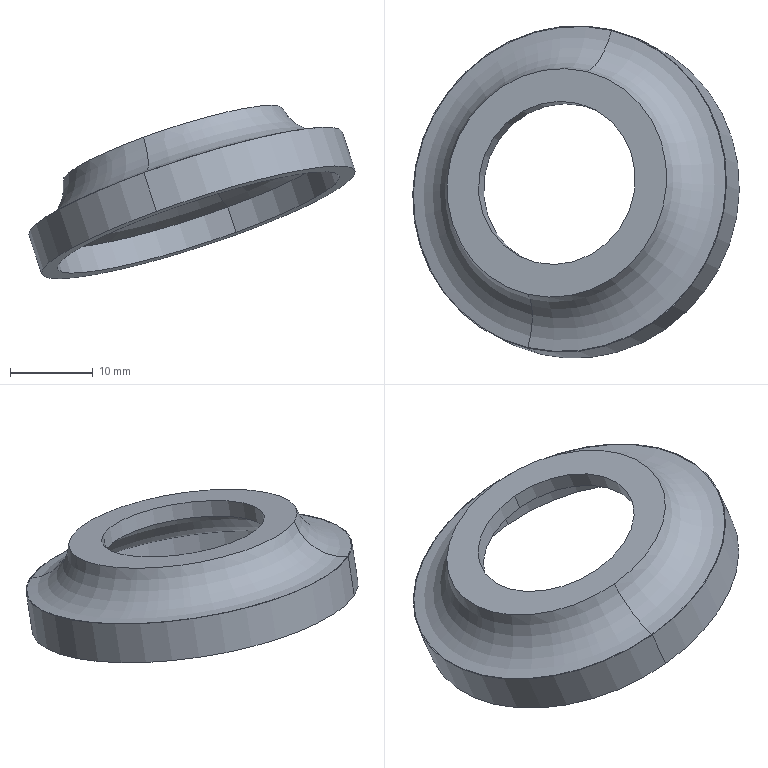Component | SolidWorks | FilmPressingSoilCoveringMechanism2Reverse-2_AttachedSoilDiskAssembly2-1_DustCover-1 | 1 solid | 14 faces | box 39.58 x 40.3 x 21.03 mm | volume 3029 mm3 | cylinder 6 | torus 4 | plane 4 | commonest cylinder face diameters 20 x2 36 x2 40 x2
STEP:
#1=COLOUR_RGB('',0.7922,0.8196,0.9333);
#2=FILL_AREA_STYLE_COLOUR('',#1);
#3=FILL_AREA_STYLE('',(#2));
#4=SURFACE_STYLE_FILL_AREA(#3);
#5=SURFACE_SIDE_STYLE('',(#4));
#6=SURFACE_STYLE_USAGE(.BOTH.,#5);
#7=PRESENTATION_STYLE_ASSIGNMENT((#6));
#8=CARTESIAN_POINT('',(-76.149,-11.265,104.072));
#9=VERTEX_POINT('',#8);
#10=CARTESIAN_POINT('',(-76.349,-12.025,104.124));
#11=VERTEX_POINT('',#10);
#12=CARTESIAN_POINT('',(-76.249,-11.645,104.098));
#13=DIRECTION('',(-0.3093,0.1459,0.9397));
#14=DIRECTION('',(-0.2542,-0.9649,0.06614));
#15=AXIS2_PLACEMENT_3D('',#12,#13,#14);
#16=CIRCLE('',#15,0.3937);
#17=EDGE_CURVE('',#9,#11,#16,.T.);
#18=ORIENTED_EDGE('',*,*,#17,.F.);
#19=CARTESIAN_POINT('',(-76.173,-11.254,104.146));
#20=VERTEX_POINT('',#19);
#21=CARTESIAN_POINT('',(-76.027,-11.323,103.702));
#22=DIRECTION('',(-0.3093,0.1459,0.9397));
#23=VECTOR('',#22,39.37);
#24=LINE('',#21,#23);
#25=EDGE_CURVE('',#9,#20,#24,.T.);
#26=ORIENTED_EDGE('',*,*,#25,.T.);
#27=CARTESIAN_POINT('',(-76.374,-12.013,104.198));
#28=VERTEX_POINT('',#27);
#29=CARTESIAN_POINT('',(-76.273,-11.634,104.172));
#30=DIRECTION('',(-0.3093,0.1459,0.9397));
#31=DIRECTION('',(-0.2542,-0.9649,0.06614));
#32=AXIS2_PLACEMENT_3D('',#29,#30,#31);
#33=CIRCLE('',#32,0.3937);
#34=EDGE_CURVE('',#20,#28,#33,.T.);
#35=ORIENTED_EDGE('',*,*,#34,.T.);
#36=CARTESIAN_POINT('',(-76.227,-12.082,103.754));
#37=DIRECTION('',(-0.3093,0.1459,0.9397));
#38=VECTOR('',#37,39.37);
#39=LINE('',#36,#38);
#40=EDGE_CURVE('',#11,#28,#39,.T.);
#41=ORIENTED_EDGE('',*,*,#40,.F.);
#42=EDGE_LOOP('',(#18,#26,#35,#41));
#43=FACE_OUTER_BOUND('',#42,.T.);
#44=CARTESIAN_POINT('',(-76.127,-11.703,103.728));
#45=DIRECTION('',(-0.3093,0.1459,0.9397));
#46=DIRECTION('',(-0.2542,-0.9649,0.06614));
#47=AXIS2_PLACEMENT_3D('',#44,#45,#46);
#48=CYLINDRICAL_SURFACE('',#47,0.3937);
#49=ADVANCED_FACE('',(#43),#48,.F.);
#50=CARTESIAN_POINT('',(-76.374,-12.12,104.13));
#51=VERTEX_POINT('',#50);
#52=CARTESIAN_POINT('',(-76.124,-11.17,104.065));
#53=VERTEX_POINT('',#52);
#54=CARTESIAN_POINT('',(-76.249,-11.645,104.098));
#55=DIRECTION('',(-0.3093,0.1459,0.9397));
#56=DIRECTION('',(0.2542,0.9649,-0.06614));
#57=AXIS2_PLACEMENT_3D('',#54,#55,#56);
#58=CIRCLE('',#57,0.4921);
#59=EDGE_CURVE('',#51,#53,#58,.T.);
#60=ORIENTED_EDGE('',*,*,#59,.T.);
#61=CARTESIAN_POINT('',(-76.011,-10.989,103.875));
#62=VERTEX_POINT('',#61);
#63=CARTESIAN_POINT('',(-76.086,-10.871,104.157));
#64=DIRECTION('',(0.9163,-0.2184,0.3356));
#65=DIRECTION('',(0.3439,0.,-0.939));
#66=AXIS2_PLACEMENT_3D('',#63,#64,#65);
#67=CIRCLE('',#66,0.315);
#68=EDGE_CURVE('',#53,#62,#67,.T.);
#69=ORIENTED_EDGE('',*,*,#68,.T.);
#70=CARTESIAN_POINT('',(-76.371,-12.356,103.968));
#71=VERTEX_POINT('',#70);
#72=CARTESIAN_POINT('',(-76.191,-11.672,103.922));
#73=DIRECTION('',(0.3093,-0.1459,-0.9397));
#74=DIRECTION('',(-0.2542,-0.9649,0.06614));
#75=AXIS2_PLACEMENT_3D('',#72,#73,#74);
#76=CIRCLE('',#75,0.7087);
#77=EDGE_CURVE('',#62,#71,#76,.T.);
#78=ORIENTED_EDGE('',*,*,#77,.T.);
#79=CARTESIAN_POINT('',(-76.485,-12.384,104.261));
#80=DIRECTION('',(-0.9163,0.2184,-0.3356));
#81=DIRECTION('',(-0.3439,0.,0.939));
#82=AXIS2_PLACEMENT_3D('',#79,#80,#81);
#83=CIRCLE('',#82,0.315);
#84=EDGE_CURVE('',#51,#71,#83,.T.);
#85=ORIENTED_EDGE('',*,*,#84,.F.);
#86=EDGE_LOOP('',(#60,#69,#78,#85));
#87=FACE_OUTER_BOUND('',#86,.T.);
#88=CARTESIAN_POINT('',(-76.286,-11.628,104.209));
#89=DIRECTION('',(-0.3093,0.1459,0.9397));
#90=DIRECTION('',(-0.2542,-0.9649,0.06614));
#91=AXIS2_PLACEMENT_3D('',#88,#89,#90);
#92=TOROIDAL_SURFACE('',#91,0.7841,0.315);
#93=ADVANCED_FACE('',(#87),#92,.T.);
#94=CARTESIAN_POINT('',(-76.191,-11.672,103.922));
#95=DIRECTION('',(0.3093,-0.1459,-0.9397));
#96=DIRECTION('',(-0.2542,-0.9649,0.06614));
#97=AXIS2_PLACEMENT_3D('',#94,#95,#96);
#98=CIRCLE('',#97,0.7087);
#99=EDGE_CURVE('',#71,#62,#98,.T.);
#100=ORIENTED_EDGE('',*,*,#99,.F.);
#101=CARTESIAN_POINT('',(-76.332,-12.375,103.849));
#102=VERTEX_POINT('',#101);
#103=CARTESIAN_POINT('',(-76.393,-12.346,104.034));
#104=DIRECTION('',(0.3093,-0.1459,-0.9397));
#105=VECTOR('',#104,39.37);
#106=LINE('',#103,#105);
#107=EDGE_CURVE('',#71,#102,#106,.T.);
#108=ORIENTED_EDGE('',*,*,#107,.T.);
#109=CARTESIAN_POINT('',(-75.972,-11.007,103.755));
#110=VERTEX_POINT('',#109);
#111=CARTESIAN_POINT('',(-76.152,-11.691,103.802));
#112=DIRECTION('',(-0.3093,0.1459,0.9397));
#113=DIRECTION('',(-0.2542,-0.9649,0.06614));
#114=AXIS2_PLACEMENT_3D('',#111,#112,#113);
#115=CIRCLE('',#114,0.7087);
#116=EDGE_CURVE('',#110,#102,#115,.T.);
#117=ORIENTED_EDGE('',*,*,#116,.F.);
#118=CARTESIAN_POINT('',(-76.032,-10.979,103.94));
#119=DIRECTION('',(0.3093,-0.1459,-0.9397));
#120=VECTOR('',#119,39.37);
#121=LINE('',#118,#120);
#122=EDGE_CURVE('',#62,#110,#121,.T.);
#123=ORIENTED_EDGE('',*,*,#122,.F.);
#124=EDGE_LOOP('',(#100,#108,#117,#123));
#125=FACE_OUTER_BOUND('',#124,.T.);
#126=CARTESIAN_POINT('',(-76.213,-11.662,103.987));
#127=DIRECTION('',(0.3093,-0.1459,-0.9397));
#128=DIRECTION('',(0.2542,0.9649,-0.06614));
#129=AXIS2_PLACEMENT_3D('',#126,#127,#128);
#130=CYLINDRICAL_SURFACE('',#129,0.7087);
#131=ADVANCED_FACE('',(#125),#130,.F.);
#132=CARTESIAN_POINT('',(-76.133,-11.102,104.135));
#133=VERTEX_POINT('',#132);
#134=CARTESIAN_POINT('',(-76.414,-12.165,104.208));
#135=VERTEX_POINT('',#134);
#136=CARTESIAN_POINT('',(-76.273,-11.634,104.172));
#137=DIRECTION('',(-0.3093,0.1459,0.9397));
#138=DIRECTION('',(-0.2542,-0.9649,0.06614));
#139=AXIS2_PLACEMENT_3D('',#136,#137,#138);
#140=CIRCLE('',#139,0.5512);
#141=EDGE_CURVE('',#133,#135,#140,.T.);
#142=ORIENTED_EDGE('',*,*,#141,.F.);
#143=CARTESIAN_POINT('',(-76.013,-10.906,103.935));
#144=VERTEX_POINT('',#143);
#145=CARTESIAN_POINT('',(-76.086,-10.871,104.157));
#146=DIRECTION('',(0.9163,-0.2184,0.3356));
#147=DIRECTION('',(0.3439,0.,-0.939));
#148=AXIS2_PLACEMENT_3D('',#145,#146,#147);
#149=CIRCLE('',#148,0.2362);
#150=EDGE_CURVE('',#133,#144,#149,.T.);
#151=ORIENTED_EDGE('',*,*,#150,.T.);
#152=CARTESIAN_POINT('',(-76.412,-12.419,104.039));
#153=VERTEX_POINT('',#152);
#154=CARTESIAN_POINT('',(-76.213,-11.662,103.987));
#155=DIRECTION('',(0.3093,-0.1459,-0.9397));
#156=DIRECTION('',(-0.2542,-0.9649,0.06614));
#157=AXIS2_PLACEMENT_3D('',#154,#155,#156);
#158=CIRCLE('',#157,0.7841);
#159=EDGE_CURVE('',#153,#144,#158,.T.);
#160=ORIENTED_EDGE('',*,*,#159,.F.);
#161=CARTESIAN_POINT('',(-76.485,-12.384,104.261));
#162=DIRECTION('',(-0.9163,0.2184,-0.3356));
#163=DIRECTION('',(-0.3439,0.,0.939));
#164=AXIS2_PLACEMENT_3D('',#161,#162,#163);
#165=CIRCLE('',#164,0.2362);
#166=EDGE_CURVE('',#135,#153,#165,.T.);
#167=ORIENTED_EDGE('',*,*,#166,.F.);
#168=EDGE_LOOP('',(#142,#151,#160,#167));
#169=FACE_OUTER_BOUND('',#168,.T.);
#170=CARTESIAN_POINT('',(-76.286,-11.628,104.209));
#171=DIRECTION('',(-0.3093,0.1459,0.9397));
#172=DIRECTION('',(-0.2542,-0.9649,0.06614));
#173=AXIS2_PLACEMENT_3D('',#170,#171,#172);
#174=TOROIDAL_SURFACE('',#173,0.7841,0.2362);
#175=ADVANCED_FACE('',(#169),#174,.F.);
#176=CARTESIAN_POINT('',(-76.413,-12.422,104.039));
#177=VERTEX_POINT('',#176);
#178=CARTESIAN_POINT('',(-76.012,-10.903,103.935));
#179=VERTEX_POINT('',#178);
#180=CARTESIAN_POINT('',(-76.213,-11.662,103.987));
#181=DIRECTION('',(-0.3093,0.1459,0.9397));
#182=DIRECTION('',(-0.2542,-0.9649,0.06614));
#183=AXIS2_PLACEMENT_3D('',#180,#181,#182);
#184=CIRCLE('',#183,0.7874);
#185=EDGE_CURVE('',#177,#179,#184,.T.);
#186=ORIENTED_EDGE('',*,*,#185,.F.);
#187=CARTESIAN_POINT('',(-76.352,-12.451,103.854));
#188=VERTEX_POINT('',#187);
#189=CARTESIAN_POINT('',(-76.413,-12.422,104.039));
#190=DIRECTION('',(0.3093,-0.1459,-0.9397));
#191=VECTOR('',#190,39.37);
#192=LINE('',#189,#191);
#193=EDGE_CURVE('',#177,#188,#192,.T.);
#194=ORIENTED_EDGE('',*,*,#193,.T.);
#195=CARTESIAN_POINT('',(-75.952,-10.931,103.75));
#196=VERTEX_POINT('',#195);
#197=CARTESIAN_POINT('',(-76.152,-11.691,103.802));
#198=DIRECTION('',(-0.3093,0.1459,0.9397));
#199=DIRECTION('',(-0.2542,-0.9649,0.06614));
#200=AXIS2_PLACEMENT_3D('',#197,#198,#199);
#201=CIRCLE('',#200,0.7874);
#202=EDGE_CURVE('',#188,#196,#201,.T.);
#203=ORIENTED_EDGE('',*,*,#202,.T.);
#204=CARTESIAN_POINT('',(-76.012,-10.903,103.935));
#205=DIRECTION('',(0.3093,-0.1459,-0.9397));
#206=VECTOR('',#205,39.37);
#207=LINE('',#204,#206);
#208=EDGE_CURVE('',#179,#196,#207,.T.);
#209=ORIENTED_EDGE('',*,*,#208,.F.);
#210=EDGE_LOOP('',(#186,#194,#203,#209));
#211=FACE_OUTER_BOUND('',#210,.T.);
#212=CARTESIAN_POINT('',(-76.213,-11.662,103.987));
#213=DIRECTION('',(0.3093,-0.1459,-0.9397));
#214=DIRECTION('',(0.2542,0.9649,-0.06614));
#215=AXIS2_PLACEMENT_3D('',#212,#213,#214);
#216=CYLINDRICAL_SURFACE('',#215,0.7874);
#217=ADVANCED_FACE('',(#211),#216,.T.);
#218=ORIENTED_EDGE('',*,*,#159,.T.);
#219=CARTESIAN_POINT('',(-76.213,-11.662,103.987));
#220=DIRECTION('',(0.3093,-0.1459,-0.9397));
#221=DIRECTION('',(-0.2542,-0.9649,0.06614));
#222=AXIS2_PLACEMENT_3D('',#219,#220,#221);
#223=CIRCLE('',#222,0.7841);
#224=EDGE_CURVE('',#144,#153,#223,.T.);
#225=ORIENTED_EDGE('',*,*,#224,.T.);
#226=EDGE_LOOP('',(#218,#225));
#227=FACE_BOUND('',#226,.T.);
#228=CARTESIAN_POINT('',(-76.213,-11.662,103.987));
#229=DIRECTION('',(-0.3093,0.1459,0.9397));
#230=DIRECTION('',(-0.2542,-0.9649,0.06614));
#231=AXIS2_PLACEMENT_3D('',#228,#229,#230);
#232=CIRCLE('',#231,0.7874);
#233=EDGE_CURVE('',#179,#177,#232,.T.);
#234=ORIENTED_EDGE('',*,*,#233,.T.);
#235=ORIENTED_EDGE('',*,*,#185,.T.);
#236=EDGE_LOOP('',(#234,#235));
#237=FACE_OUTER_BOUND('',#236,.T.);
#238=CARTESIAN_POINT('',(-76.213,-11.662,103.987));
#239=DIRECTION('',(-0.3093,0.1459,0.9397));
#240=DIRECTION('',(-0.2542,-0.9649,0.06614));
#241=AXIS2_PLACEMENT_3D('',#238,#239,#240);
#242=PLANE('',#241);
#243=ADVANCED_FACE('',(#227,#237),#242,.T.);
#244=ORIENTED_EDGE('',*,*,#193,.F.);
#245=ORIENTED_EDGE('',*,*,#233,.F.);
#246=ORIENTED_EDGE('',*,*,#208,.T.);
#247=CARTESIAN_POINT('',(-76.152,-11.691,103.802));
#248=DIRECTION('',(-0.3093,0.1459,0.9397));
#249=DIRECTION('',(-0.2542,-0.9649,0.06614));
#250=AXIS2_PLACEMENT_3D('',#247,#248,#249);
#251=CIRCLE('',#250,0.7874);
#252=EDGE_CURVE('',#196,#188,#251,.T.);
#253=ORIENTED_EDGE('',*,*,#252,.T.);
#254=EDGE_LOOP('',(#244,#245,#246,#253));
#255=FACE_OUTER_BOUND('',#254,.T.);
#256=CARTESIAN_POINT('',(-76.213,-11.662,103.987));
#257=DIRECTION('',(0.3093,-0.1459,-0.9397));
#258=DIRECTION('',(0.2542,0.9649,-0.06614));
#259=AXIS2_PLACEMENT_3D('',#256,#257,#258);
#260=CYLINDRICAL_SURFACE('',#259,0.7874);
#261=ADVANCED_FACE('',(#255),#260,.T.);
#262=ORIENTED_EDGE('',*,*,#116,.T.);
#263=CARTESIAN_POINT('',(-76.152,-11.691,103.802));
#264=DIRECTION('',(-0.3093,0.1459,0.9397));
#265=DIRECTION('',(-0.2542,-0.9649,0.06614));
#266=AXIS2_PLACEMENT_3D('',#263,#264,#265);
#267=CIRCLE('',#266,0.7087);
#268=EDGE_CURVE('',#102,#110,#267,.T.);
#269=ORIENTED_EDGE('',*,*,#268,.T.);
#270=EDGE_LOOP('',(#262,#269));
#271=FACE_BOUND('',#270,.T.);
#272=ORIENTED_EDGE('',*,*,#252,.F.);
#273=ORIENTED_EDGE('',*,*,#202,.F.);
#274=EDGE_LOOP('',(#272,#273));
#275=FACE_OUTER_BOUND('',#274,.T.);
#276=CARTESIAN_POINT('',(-76.152,-11.691,103.802));
#277=DIRECTION('',(-0.3093,0.1459,0.9397));
#278=DIRECTION('',(-0.2542,-0.9649,0.06614));
#279=AXIS2_PLACEMENT_3D('',#276,#277,#278);
#280=PLANE('',#279);
#281=ADVANCED_FACE('',(#271,#275),#280,.F.);
#282=CARTESIAN_POINT('',(-76.273,-11.634,104.172));
#283=DIRECTION('',(-0.3093,0.1459,0.9397));
#284=DIRECTION('',(-0.2542,-0.9649,0.06614));
#285=AXIS2_PLACEMENT_3D('',#282,#283,#284);
#286=CIRCLE('',#285,0.3937);
#287=EDGE_CURVE('',#28,#20,#286,.T.);
#288=ORIENTED_EDGE('',*,*,#287,.F.);
#289=ORIENTED_EDGE('',*,*,#34,.F.);
#290=EDGE_LOOP('',(#288,#289));
#291=FACE_BOUND('',#290,.T.);
#292=CARTESIAN_POINT('',(-76.273,-11.634,104.172));
#293=DIRECTION('',(-0.3093,0.1459,0.9397));
#294=DIRECTION('',(-0.2542,-0.9649,0.06614));
#295=AXIS2_PLACEMENT_3D('',#292,#293,#294);
#296=CIRCLE('',#295,0.5512);
#297=EDGE_CURVE('',#135,#133,#296,.T.);
#298=ORIENTED_EDGE('',*,*,#297,.T.);
#299=ORIENTED_EDGE('',*,*,#141,.T.);
#300=EDGE_LOOP('',(#298,#299));
#301=FACE_OUTER_BOUND('',#300,.T.);
#302=CARTESIAN_POINT('',(-76.273,-11.634,104.172));
#303=DIRECTION('',(-0.3093,0.1459,0.9397));
#304=DIRECTION('',(-0.2542,-0.9649,0.06614));
#305=AXIS2_PLACEMENT_3D('',#302,#303,#304);
#306=PLANE('',#305);
#307=ADVANCED_FACE('',(#291,#301),#306,.T.);
#308=ORIENTED_EDGE('',*,*,#150,.F.);
#309=ORIENTED_EDGE('',*,*,#297,.F.);
#310=ORIENTED_EDGE('',*,*,#166,.T.);
#311=ORIENTED_EDGE('',*,*,#224,.F.);
#312=EDGE_LOOP('',(#308,#309,#310,#311));
#313=FACE_OUTER_BOUND('',#312,.T.);
#314=CARTESIAN_POINT('',(-76.286,-11.628,104.209));
#315=DIRECTION('',(-0.3093,0.1459,0.9397));
#316=DIRECTION('',(-0.2542,-0.9649,0.06614));
#317=AXIS2_PLACEMENT_3D('',#314,#315,#316);
#318=TOROIDAL_SURFACE('',#317,0.7841,0.2362);
#319=ADVANCED_FACE('',(#313),#318,.F.);
#320=ORIENTED_EDGE('',*,*,#107,.F.);
#321=ORIENTED_EDGE('',*,*,#77,.F.);
#322=ORIENTED_EDGE('',*,*,#122,.T.);
#323=ORIENTED_EDGE('',*,*,#268,.F.);
#324=EDGE_LOOP('',(#320,#321,#322,#323));
#325=FACE_OUTER_BOUND('',#324,.T.);
#326=CARTESIAN_POINT('',(-76.213,-11.662,103.987));
#327=DIRECTION('',(0.3093,-0.1459,-0.9397));
#328=DIRECTION('',(0.2542,0.9649,-0.06614));
#329=AXIS2_PLACEMENT_3D('',#326,#327,#328);
#330=CYLINDRICAL_SURFACE('',#329,0.7087);
#331=ADVANCED_FACE('',(#325),#330,.F.);
#332=CARTESIAN_POINT('',(-76.249,-11.645,104.098));
#333=DIRECTION('',(-0.3093,0.1459,0.9397));
#334=DIRECTION('',(-0.2542,-0.9649,0.06614));
#335=AXIS2_PLACEMENT_3D('',#332,#333,#334);
#336=CIRCLE('',#335,0.3937);
#337=EDGE_CURVE('',#11,#9,#336,.T.);
#338=ORIENTED_EDGE('',*,*,#337,.T.);
#339=ORIENTED_EDGE('',*,*,#17,.T.);
#340=EDGE_LOOP('',(#338,#339));
#341=FACE_BOUND('',#340,.T.);
#342=ORIENTED_EDGE('',*,*,#59,.F.);
#343=CARTESIAN_POINT('',(-76.249,-11.645,104.098));
#344=DIRECTION('',(-0.3093,0.1459,0.9397));
#345=DIRECTION('',(0.2542,0.9649,-0.06614));
#346=AXIS2_PLACEMENT_3D('',#343,#344,#345);
#347=CIRCLE('',#346,0.4921);
#348=EDGE_CURVE('',#53,#51,#347,.T.);
#349=ORIENTED_EDGE('',*,*,#348,.F.);
#350=EDGE_LOOP('',(#342,#349));
#351=FACE_OUTER_BOUND('',#350,.T.);
#352=CARTESIAN_POINT('',(-76.249,-11.645,104.098));
#353=DIRECTION('',(-0.3093,0.1459,0.9397));
#354=DIRECTION('',(-0.2542,-0.9649,0.06614));
#355=AXIS2_PLACEMENT_3D('',#352,#353,#354);
#356=PLANE('',#355);
#357=ADVANCED_FACE('',(#341,#351),#356,.F.);
#358=ORIENTED_EDGE('',*,*,#68,.F.);
#359=ORIENTED_EDGE('',*,*,#348,.T.);
#360=ORIENTED_EDGE('',*,*,#84,.T.);
#361=ORIENTED_EDGE('',*,*,#99,.T.);
#362=EDGE_LOOP('',(#358,#359,#360,#361));
#363=FACE_OUTER_BOUND('',#362,.T.);
#364=CARTESIAN_POINT('',(-76.286,-11.628,104.209));
#365=DIRECTION('',(-0.3093,0.1459,0.9397));
#366=DIRECTION('',(-0.2542,-0.9649,0.06614));
#367=AXIS2_PLACEMENT_3D('',#364,#365,#366);
#368=TOROIDAL_SURFACE('',#367,0.7841,0.315);
#369=ADVANCED_FACE('',(#363),#368,.T.);
#370=ORIENTED_EDGE('',*,*,#25,.F.);
#371=ORIENTED_EDGE('',*,*,#337,.F.);
#372=ORIENTED_EDGE('',*,*,#40,.T.);
#373=ORIENTED_EDGE('',*,*,#287,.T.);
#374=EDGE_LOOP('',(#370,#371,#372,#373));
#375=FACE_OUTER_BOUND('',#374,.T.);
#376=CARTESIAN_POINT('',(-76.127,-11.703,103.728));
#377=DIRECTION('',(-0.3093,0.1459,0.9397));
#378=DIRECTION('',(-0.2542,-0.9649,0.06614));
#379=AXIS2_PLACEMENT_3D('',#376,#377,#378);
#380=CYLINDRICAL_SURFACE('',#379,0.3937);
#381=ADVANCED_FACE('',(#375),#380,.F.);
#382=CLOSED_SHELL('',(#49,#93,#131,#175,#217,#243,#261,#281,#307,#319,#331,#357,#369,#381));
#383=MANIFOLD_SOLID_BREP('',#382);
#384=STYLED_ITEM('',(#7),#383);
#385=(LENGTH_UNIT()NAMED_UNIT(*)SI_UNIT($,.METRE.));
#386=LENGTH_MEASURE_WITH_UNIT(LENGTH_MEASURE(0.0254),#385);
#387=DIMENSIONAL_EXPONENTS(1.,0.,0.,0.,0.,0.,0.);
#388=(CONVERSION_BASED_UNIT('',#386)LENGTH_UNIT()NAMED_UNIT(#387));
#389=UNCERTAINTY_MEASURE_WITH_UNIT(LENGTH_MEASURE(0.00001),#388,'','');
#390=(NAMED_UNIT(*)PLANE_ANGLE_UNIT()SI_UNIT($,.RADIAN.));
#391=(NAMED_UNIT(*)SI_UNIT($,.STERADIAN.)SOLID_ANGLE_UNIT());
#392=(GEOMETRIC_REPRESENTATION_CONTEXT(3)GLOBAL_UNCERTAINTY_ASSIGNED_CONTEXT((#389))GLOBAL_UNIT_ASSIGNED_CONTEXT((#388,#390,#391))REPRESENTATION_CONTEXT('',''));
#393=MECHANICAL_DESIGN_GEOMETRIC_PRESENTATION_REPRESENTATION('',(#384),#392);
#394=PRESENTATION_LAYER_ASSIGNMENT('','',(#384));
#395=CARTESIAN_POINT('',(0.,0.,0.));
#396=DIRECTION('',(0.,0.,1.));
#397=DIRECTION('',(1.,0.,0.));
#398=AXIS2_PLACEMENT_3D('',#395,#396,#397);
#399=(LENGTH_UNIT()NAMED_UNIT(*)SI_UNIT($,.METRE.));
#400=LENGTH_MEASURE_WITH_UNIT(LENGTH_MEASURE(0.0254),#399);
#401=DIMENSIONAL_EXPONENTS(1.,0.,0.,0.,0.,0.,0.);
#402=(CONVERSION_BASED_UNIT('',#400)LENGTH_UNIT()NAMED_UNIT(#401));
#403=UNCERTAINTY_MEASURE_WITH_UNIT(LENGTH_MEASURE(0.00001),#402,'','');
#404=(NAMED_UNIT(*)PLANE_ANGLE_UNIT()SI_UNIT($,.RADIAN.));
#405=(NAMED_UNIT(*)SI_UNIT($,.STERADIAN.)SOLID_ANGLE_UNIT());
#406=(GEOMETRIC_REPRESENTATION_CONTEXT(3)GLOBAL_UNCERTAINTY_ASSIGNED_CONTEXT((#403))GLOBAL_UNIT_ASSIGNED_CONTEXT((#402,#404,#405))REPRESENTATION_CONTEXT('',''));
#407=ADVANCED_BREP_SHAPE_REPRESENTATION('',(#383,#398),#406);